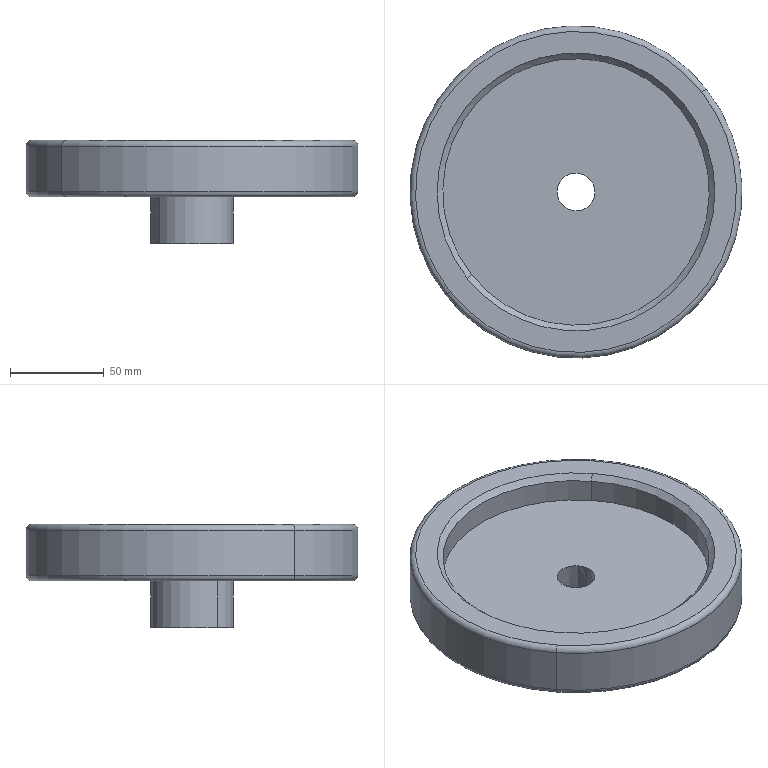Component | SolidWorks | 3-1 | 1 solid | 18 faces | box 177 x 177 x 55 mm | volume 506680 mm3 | cylinder 6 | cone 4 | torus 4 | plane 4 | commonest cylinder face diameters 177 x2 44 x2 142 x2
build123d program:
from build123d import *

# Parameters (mm, degrees)
CHAMFER1_SIZE = 3


with BuildPart() as part:
    # Sketch1 → Revolve1 (revolve)
    with BuildSketch(Plane(origin=(0, 0, 0), x_dir=(1, 0, 0), z_dir=(0, 1, 0))):
        with BuildLine():
            Line((0, 85.5), (0, 71))
            Line((0, 71), (15.508, 71))
            Line((15.508, 71), (15.508, 10.064))
            Line((15.508, 10.064), (55, 15))
            Line((55, 15), (55, 22))
            Line((55, 22), (30, 22))
            Line((30, 22), (30, 85.5))
            ThreePointArc((30, 85.5), (29.121, 87.621), (27, 88.5))
            Line((27, 88.5), (3, 88.5))
            ThreePointArc((3, 88.5), (0.8787, 87.621), (0, 85.5))
        make_face()
    revolve(axis=Axis((55, 0, 0), (-1, 0, 0)))

    # Chamfer1
    chamfer1_edges = [part.edges().sort_by_distance(p)[0] for p in [
        (0, 0, 71),
    ]]
    chamfer(chamfer1_edges, length=CHAMFER1_SIZE)


solid = part.part

# Placed as in the assembly
solid = solid.moved(Location((-135.043, 380.991, 857.751), (0, 90, 0)))
STEP:
#1=COLOUR_RGB('',0.7922,0.8196,0.9333);
#2=FILL_AREA_STYLE_COLOUR('',#1);
#3=FILL_AREA_STYLE('',(#2));
#4=SURFACE_STYLE_FILL_AREA(#3);
#5=SURFACE_SIDE_STYLE('',(#4));
#6=SURFACE_STYLE_USAGE(.BOTH.,#5);
#7=PRESENTATION_STYLE_ASSIGNMENT((#6));
#8=CARTESIAN_POINT('',(-7.51,13.267,33.652));
#9=VERTEX_POINT('',#8);
#10=CARTESIAN_POINT('',(-3.123,16.732,33.652));
#11=VERTEX_POINT('',#10);
#12=CARTESIAN_POINT('',(-5.317,15.,33.652));
#13=DIRECTION('',(0.,0.,1.));
#14=DIRECTION('',(-0.7848,-0.6197,0.));
#15=AXIS2_PLACEMENT_3D('',#12,#13,#14);
#16=CIRCLE('',#15,2.795);
#17=EDGE_CURVE('',#9,#11,#16,.T.);
#18=ORIENTED_EDGE('',*,*,#17,.F.);
#19=CARTESIAN_POINT('',(-7.603,13.194,33.77));
#20=VERTEX_POINT('',#19);
#21=CARTESIAN_POINT('',(-7.603,13.194,33.77));
#22=DIRECTION('',(-0.5549,-0.4382,0.7071));
#23=VECTOR('',#22,39.37);
#24=LINE('',#21,#23);
#25=EDGE_CURVE('',#9,#20,#24,.T.);
#26=ORIENTED_EDGE('',*,*,#25,.T.);
#27=CARTESIAN_POINT('',(-3.03,16.805,33.77));
#28=VERTEX_POINT('',#27);
#29=CARTESIAN_POINT('',(-5.317,15.,33.77));
#30=DIRECTION('',(-0.,-0.,-1.));
#31=DIRECTION('',(-0.7848,-0.6197,0.));
#32=AXIS2_PLACEMENT_3D('',#29,#30,#31);
#33=CIRCLE('',#32,2.913);
#34=EDGE_CURVE('',#28,#20,#33,.T.);
#35=ORIENTED_EDGE('',*,*,#34,.F.);
#36=CARTESIAN_POINT('',(-3.03,16.805,33.77));
#37=DIRECTION('',(0.5549,0.4382,0.7071));
#38=VECTOR('',#37,39.37);
#39=LINE('',#36,#38);
#40=EDGE_CURVE('',#11,#28,#39,.T.);
#41=ORIENTED_EDGE('',*,*,#40,.F.);
#42=EDGE_LOOP('',(#18,#26,#35,#41));
#43=FACE_OUTER_BOUND('',#42,.T.);
#44=CARTESIAN_POINT('',(-5.317,15.,33.77));
#45=DIRECTION('',(0.,0.,1.));
#46=DIRECTION('',(0.7848,0.6197,0.));
#47=AXIS2_PLACEMENT_3D('',#44,#45,#46);
#48=CONICAL_SURFACE('',#47,2.913,0.7854);
#49=ADVANCED_FACE('',(#43),#48,.F.);
#50=CARTESIAN_POINT('',(-8.051,12.84,33.652));
#51=VERTEX_POINT('',#50);
#52=CARTESIAN_POINT('',(-2.582,17.159,33.652));
#53=VERTEX_POINT('',#52);
#54=CARTESIAN_POINT('',(-5.317,15.,33.652));
#55=DIRECTION('',(-0.,-0.,-1.));
#56=DIRECTION('',(-0.7848,-0.6197,0.));
#57=AXIS2_PLACEMENT_3D('',#54,#55,#56);
#58=CIRCLE('',#57,3.484);
#59=EDGE_CURVE('',#51,#53,#58,.T.);
#60=ORIENTED_EDGE('',*,*,#59,.T.);
#61=CARTESIAN_POINT('',(-2.582,17.159,32.707));
#62=VERTEX_POINT('',#61);
#63=CARTESIAN_POINT('',(-2.582,17.159,31.604));
#64=DIRECTION('',(-0.,-0.,-1.));
#65=VECTOR('',#64,39.37);
#66=LINE('',#63,#65);
#67=EDGE_CURVE('',#53,#62,#66,.T.);
#68=ORIENTED_EDGE('',*,*,#67,.T.);
#69=CARTESIAN_POINT('',(-8.051,12.84,32.707));
#70=VERTEX_POINT('',#69);
#71=CARTESIAN_POINT('',(-5.317,15.,32.707));
#72=DIRECTION('',(-0.,-0.,-1.));
#73=DIRECTION('',(-0.7848,-0.6197,0.));
#74=AXIS2_PLACEMENT_3D('',#71,#72,#73);
#75=CIRCLE('',#74,3.484);
#76=EDGE_CURVE('',#70,#62,#75,.T.);
#77=ORIENTED_EDGE('',*,*,#76,.F.);
#78=CARTESIAN_POINT('',(-8.051,12.84,31.604));
#79=DIRECTION('',(-0.,-0.,-1.));
#80=VECTOR('',#79,39.37);
#81=LINE('',#78,#80);
#82=EDGE_CURVE('',#51,#70,#81,.T.);
#83=ORIENTED_EDGE('',*,*,#82,.F.);
#84=EDGE_LOOP('',(#60,#68,#77,#83));
#85=FACE_OUTER_BOUND('',#84,.T.);
#86=CARTESIAN_POINT('',(-5.317,15.,31.604));
#87=DIRECTION('',(-0.,-0.,-1.));
#88=DIRECTION('',(-0.7848,-0.6197,0.));
#89=AXIS2_PLACEMENT_3D('',#86,#87,#88);
#90=CYLINDRICAL_SURFACE('',#89,3.484);
#91=ADVANCED_FACE('',(#85),#90,.T.);
#92=ORIENTED_EDGE('',*,*,#76,.T.);
#93=CARTESIAN_POINT('',(-2.675,17.086,32.589));
#94=VERTEX_POINT('',#93);
#95=CARTESIAN_POINT('',(-2.675,17.086,32.707));
#96=DIRECTION('',(-0.6197,0.7848,-0.));
#97=DIRECTION('',(-0.7848,-0.6197,0.));
#98=AXIS2_PLACEMENT_3D('',#95,#96,#97);
#99=CIRCLE('',#98,0.1181);
#100=EDGE_CURVE('',#62,#94,#99,.T.);
#101=ORIENTED_EDGE('',*,*,#100,.T.);
#102=CARTESIAN_POINT('',(-7.958,12.914,32.589));
#103=VERTEX_POINT('',#102);
#104=CARTESIAN_POINT('',(-5.317,15.,32.589));
#105=DIRECTION('',(-0.,-0.,-1.));
#106=DIRECTION('',(-0.7848,-0.6197,0.));
#107=AXIS2_PLACEMENT_3D('',#104,#105,#106);
#108=CIRCLE('',#107,3.366);
#109=EDGE_CURVE('',#103,#94,#108,.T.);
#110=ORIENTED_EDGE('',*,*,#109,.F.);
#111=CARTESIAN_POINT('',(-7.958,12.914,32.707));
#112=DIRECTION('',(0.6197,-0.7848,0.));
#113=DIRECTION('',(0.7848,0.6197,0.));
#114=AXIS2_PLACEMENT_3D('',#111,#112,#113);
#115=CIRCLE('',#114,0.1181);
#116=EDGE_CURVE('',#70,#103,#115,.T.);
#117=ORIENTED_EDGE('',*,*,#116,.F.);
#118=EDGE_LOOP('',(#92,#101,#110,#117));
#119=FACE_OUTER_BOUND('',#118,.T.);
#120=CARTESIAN_POINT('',(-5.317,15.,32.707));
#121=DIRECTION('',(-0.,-0.,-1.));
#122=DIRECTION('',(-0.7848,-0.6197,0.));
#123=AXIS2_PLACEMENT_3D('',#120,#121,#122);
#124=TOROIDAL_SURFACE('',#123,3.366,0.1181);
#125=ADVANCED_FACE('',(#119),#124,.T.);
#126=CARTESIAN_POINT('',(-5.996,14.463,32.589));
#127=VERTEX_POINT('',#126);
#128=CARTESIAN_POINT('',(-4.637,15.536,32.589));
#129=VERTEX_POINT('',#128);
#130=CARTESIAN_POINT('',(-5.317,15.,32.589));
#131=DIRECTION('',(-0.,-0.,-1.));
#132=DIRECTION('',(-0.7848,-0.6197,0.));
#133=AXIS2_PLACEMENT_3D('',#130,#131,#132);
#134=CIRCLE('',#133,0.8661);
#135=EDGE_CURVE('',#127,#129,#134,.T.);
#136=ORIENTED_EDGE('',*,*,#135,.T.);
#137=CARTESIAN_POINT('',(-4.637,15.536,31.604));
#138=VERTEX_POINT('',#137);
#139=CARTESIAN_POINT('',(-4.637,15.536,31.604));
#140=DIRECTION('',(-0.,-0.,-1.));
#141=VECTOR('',#140,39.37);
#142=LINE('',#139,#141);
#143=EDGE_CURVE('',#129,#138,#142,.T.);
#144=ORIENTED_EDGE('',*,*,#143,.T.);
#145=CARTESIAN_POINT('',(-5.996,14.463,31.604));
#146=VERTEX_POINT('',#145);
#147=CARTESIAN_POINT('',(-5.317,15.,31.604));
#148=DIRECTION('',(-0.,-0.,-1.));
#149=DIRECTION('',(-0.7848,-0.6197,0.));
#150=AXIS2_PLACEMENT_3D('',#147,#148,#149);
#151=CIRCLE('',#150,0.8661);
#152=EDGE_CURVE('',#146,#138,#151,.T.);
#153=ORIENTED_EDGE('',*,*,#152,.F.);
#154=CARTESIAN_POINT('',(-5.996,14.463,31.604));
#155=DIRECTION('',(-0.,-0.,-1.));
#156=VECTOR('',#155,39.37);
#157=LINE('',#154,#156);
#158=EDGE_CURVE('',#127,#146,#157,.T.);
#159=ORIENTED_EDGE('',*,*,#158,.F.);
#160=EDGE_LOOP('',(#136,#144,#153,#159));
#161=FACE_OUTER_BOUND('',#160,.T.);
#162=CARTESIAN_POINT('',(-5.317,15.,31.604));
#163=DIRECTION('',(-0.,-0.,-1.));
#164=DIRECTION('',(-0.7848,-0.6197,0.));
#165=AXIS2_PLACEMENT_3D('',#162,#163,#164);
#166=CYLINDRICAL_SURFACE('',#165,0.8661);
#167=ADVANCED_FACE('',(#161),#166,.T.);
#168=CARTESIAN_POINT('',(-5.006,15.245,33.159));
#169=VERTEX_POINT('',#168);
#170=CARTESIAN_POINT('',(-5.628,14.754,33.159));
#171=VERTEX_POINT('',#170);
#172=CARTESIAN_POINT('',(-5.317,15.,33.159));
#173=DIRECTION('',(-0.,-0.,-1.));
#174=DIRECTION('',(-0.7848,-0.6197,0.));
#175=AXIS2_PLACEMENT_3D('',#172,#173,#174);
#176=CIRCLE('',#175,0.3962);
#177=EDGE_CURVE('',#169,#171,#176,.T.);
#178=ORIENTED_EDGE('',*,*,#177,.F.);
#179=CARTESIAN_POINT('',(-4.853,15.366,31.604));
#180=VERTEX_POINT('',#179);
#181=CARTESIAN_POINT('',(-4.853,15.366,31.604));
#182=DIRECTION('',(0.09734,0.07687,-0.9923));
#183=VECTOR('',#182,39.37);
#184=LINE('',#181,#183);
#185=EDGE_CURVE('',#169,#180,#184,.T.);
#186=ORIENTED_EDGE('',*,*,#185,.T.);
#187=CARTESIAN_POINT('',(-5.78,14.634,31.604));
#188=VERTEX_POINT('',#187);
#189=CARTESIAN_POINT('',(-5.317,15.,31.604));
#190=DIRECTION('',(-0.,-0.,-1.));
#191=DIRECTION('',(-0.7848,-0.6197,0.));
#192=AXIS2_PLACEMENT_3D('',#189,#190,#191);
#193=CIRCLE('',#192,0.5906);
#194=EDGE_CURVE('',#180,#188,#193,.T.);
#195=ORIENTED_EDGE('',*,*,#194,.T.);
#196=CARTESIAN_POINT('',(-5.78,14.634,31.604));
#197=DIRECTION('',(-0.09734,-0.07687,-0.9923));
#198=VECTOR('',#197,39.37);
#199=LINE('',#196,#198);
#200=EDGE_CURVE('',#171,#188,#199,.T.);
#201=ORIENTED_EDGE('',*,*,#200,.F.);
#202=EDGE_LOOP('',(#178,#186,#195,#201));
#203=FACE_OUTER_BOUND('',#202,.T.);
#204=CARTESIAN_POINT('',(-5.317,15.,31.604));
#205=DIRECTION('',(-0.,-0.,-1.));
#206=DIRECTION('',(-0.7848,-0.6197,0.));
#207=AXIS2_PLACEMENT_3D('',#204,#205,#206);
#208=CONICAL_SURFACE('',#207,0.5906,0.1244);
#209=ADVANCED_FACE('',(#203),#208,.F.);
#210=ORIENTED_EDGE('',*,*,#17,.T.);
#211=CARTESIAN_POINT('',(-3.123,16.732,33.159));
#212=VERTEX_POINT('',#211);
#213=CARTESIAN_POINT('',(-3.123,16.732,31.604));
#214=DIRECTION('',(-0.,-0.,-1.));
#215=VECTOR('',#214,39.37);
#216=LINE('',#213,#215);
#217=EDGE_CURVE('',#11,#212,#216,.T.);
#218=ORIENTED_EDGE('',*,*,#217,.T.);
#219=CARTESIAN_POINT('',(-7.51,13.267,33.159));
#220=VERTEX_POINT('',#219);
#221=CARTESIAN_POINT('',(-5.317,15.,33.159));
#222=DIRECTION('',(-0.,-0.,-1.));
#223=DIRECTION('',(-0.7848,-0.6197,0.));
#224=AXIS2_PLACEMENT_3D('',#221,#222,#223);
#225=CIRCLE('',#224,2.795);
#226=EDGE_CURVE('',#212,#220,#225,.T.);
#227=ORIENTED_EDGE('',*,*,#226,.T.);
#228=CARTESIAN_POINT('',(-7.51,13.267,31.604));
#229=DIRECTION('',(-0.,-0.,-1.));
#230=VECTOR('',#229,39.37);
#231=LINE('',#228,#230);
#232=EDGE_CURVE('',#9,#220,#231,.T.);
#233=ORIENTED_EDGE('',*,*,#232,.F.);
#234=EDGE_LOOP('',(#210,#218,#227,#233));
#235=FACE_OUTER_BOUND('',#234,.T.);
#236=CARTESIAN_POINT('',(-5.317,15.,31.604));
#237=DIRECTION('',(-0.,-0.,-1.));
#238=DIRECTION('',(-0.7848,-0.6197,0.));
#239=AXIS2_PLACEMENT_3D('',#236,#237,#238);
#240=CYLINDRICAL_SURFACE('',#239,2.795);
#241=ADVANCED_FACE('',(#235),#240,.F.);
#242=CARTESIAN_POINT('',(-7.958,12.914,33.77));
#243=VERTEX_POINT('',#242);
#244=CARTESIAN_POINT('',(-2.675,17.086,33.77));
#245=VERTEX_POINT('',#244);
#246=CARTESIAN_POINT('',(-5.317,15.,33.77));
#247=DIRECTION('',(-0.,-0.,-1.));
#248=DIRECTION('',(-0.7848,-0.6197,0.));
#249=AXIS2_PLACEMENT_3D('',#246,#247,#248);
#250=CIRCLE('',#249,3.366);
#251=EDGE_CURVE('',#243,#245,#250,.T.);
#252=ORIENTED_EDGE('',*,*,#251,.T.);
#253=CARTESIAN_POINT('',(-2.675,17.086,33.652));
#254=DIRECTION('',(-0.6197,0.7848,-0.));
#255=DIRECTION('',(-0.7848,-0.6197,0.));
#256=AXIS2_PLACEMENT_3D('',#253,#254,#255);
#257=CIRCLE('',#256,0.1181);
#258=EDGE_CURVE('',#245,#53,#257,.T.);
#259=ORIENTED_EDGE('',*,*,#258,.T.);
#260=ORIENTED_EDGE('',*,*,#59,.F.);
#261=CARTESIAN_POINT('',(-7.958,12.914,33.652));
#262=DIRECTION('',(0.6197,-0.7848,0.));
#263=DIRECTION('',(0.7848,0.6197,0.));
#264=AXIS2_PLACEMENT_3D('',#261,#262,#263);
#265=CIRCLE('',#264,0.1181);
#266=EDGE_CURVE('',#243,#51,#265,.T.);
#267=ORIENTED_EDGE('',*,*,#266,.F.);
#268=EDGE_LOOP('',(#252,#259,#260,#267));
#269=FACE_OUTER_BOUND('',#268,.T.);
#270=CARTESIAN_POINT('',(-5.317,15.,33.652));
#271=DIRECTION('',(-0.,-0.,-1.));
#272=DIRECTION('',(-0.7848,-0.6197,0.));
#273=AXIS2_PLACEMENT_3D('',#270,#271,#272);
#274=TOROIDAL_SURFACE('',#273,3.366,0.1181);
#275=ADVANCED_FACE('',(#269),#274,.T.);
#276=ORIENTED_EDGE('',*,*,#258,.F.);
#277=CARTESIAN_POINT('',(-5.317,15.,33.77));
#278=DIRECTION('',(-0.,-0.,-1.));
#279=DIRECTION('',(-0.7848,-0.6197,0.));
#280=AXIS2_PLACEMENT_3D('',#277,#278,#279);
#281=CIRCLE('',#280,3.366);
#282=EDGE_CURVE('',#245,#243,#281,.T.);
#283=ORIENTED_EDGE('',*,*,#282,.T.);
#284=ORIENTED_EDGE('',*,*,#266,.T.);
#285=CARTESIAN_POINT('',(-5.317,15.,33.652));
#286=DIRECTION('',(-0.,-0.,-1.));
#287=DIRECTION('',(-0.7848,-0.6197,0.));
#288=AXIS2_PLACEMENT_3D('',#285,#286,#287);
#289=CIRCLE('',#288,3.484);
#290=EDGE_CURVE('',#53,#51,#289,.T.);
#291=ORIENTED_EDGE('',*,*,#290,.F.);
#292=EDGE_LOOP('',(#276,#283,#284,#291));
#293=FACE_OUTER_BOUND('',#292,.T.);
#294=CARTESIAN_POINT('',(-5.317,15.,33.652));
#295=DIRECTION('',(-0.,-0.,-1.));
#296=DIRECTION('',(-0.7848,-0.6197,0.));
#297=AXIS2_PLACEMENT_3D('',#294,#295,#296);
#298=TOROIDAL_SURFACE('',#297,3.366,0.1181);
#299=ADVANCED_FACE('',(#293),#298,.T.);
#300=ORIENTED_EDGE('',*,*,#34,.T.);
#301=CARTESIAN_POINT('',(-5.317,15.,33.77));
#302=DIRECTION('',(-0.,-0.,-1.));
#303=DIRECTION('',(-0.7848,-0.6197,0.));
#304=AXIS2_PLACEMENT_3D('',#301,#302,#303);
#305=CIRCLE('',#304,2.913);
#306=EDGE_CURVE('',#20,#28,#305,.T.);
#307=ORIENTED_EDGE('',*,*,#306,.T.);
#308=EDGE_LOOP('',(#300,#307));
#309=FACE_BOUND('',#308,.T.);
#310=ORIENTED_EDGE('',*,*,#251,.F.);
#311=ORIENTED_EDGE('',*,*,#282,.F.);
#312=EDGE_LOOP('',(#310,#311));
#313=FACE_OUTER_BOUND('',#312,.T.);
#314=CARTESIAN_POINT('',(-5.317,15.,33.77));
#315=DIRECTION('',(-0.,-0.,-1.));
#316=DIRECTION('',(-0.7848,-0.6197,0.));
#317=AXIS2_PLACEMENT_3D('',#314,#315,#316);
#318=PLANE('',#317);
#319=ADVANCED_FACE('',(#309,#313),#318,.F.);
#320=ORIENTED_EDGE('',*,*,#217,.F.);
#321=CARTESIAN_POINT('',(-5.317,15.,33.652));
#322=DIRECTION('',(0.,0.,1.));
#323=DIRECTION('',(-0.7848,-0.6197,0.));
#324=AXIS2_PLACEMENT_3D('',#321,#322,#323);
#325=CIRCLE('',#324,2.795);
#326=EDGE_CURVE('',#11,#9,#325,.T.);
#327=ORIENTED_EDGE('',*,*,#326,.T.);
#328=ORIENTED_EDGE('',*,*,#232,.T.);
#329=CARTESIAN_POINT('',(-5.317,15.,33.159));
#330=DIRECTION('',(-0.,-0.,-1.));
#331=DIRECTION('',(-0.7848,-0.6197,0.));
#332=AXIS2_PLACEMENT_3D('',#329,#330,#331);
#333=CIRCLE('',#332,2.795);
#334=EDGE_CURVE('',#220,#212,#333,.T.);
#335=ORIENTED_EDGE('',*,*,#334,.T.);
#336=EDGE_LOOP('',(#320,#327,#328,#335));
#337=FACE_OUTER_BOUND('',#336,.T.);
#338=CARTESIAN_POINT('',(-5.317,15.,31.604));
#339=DIRECTION('',(-0.,-0.,-1.));
#340=DIRECTION('',(-0.7848,-0.6197,0.));
#341=AXIS2_PLACEMENT_3D('',#338,#339,#340);
#342=CYLINDRICAL_SURFACE('',#341,2.795);
#343=ADVANCED_FACE('',(#337),#342,.F.);
#344=CARTESIAN_POINT('',(-5.317,15.,33.159));
#345=DIRECTION('',(-0.,-0.,-1.));
#346=DIRECTION('',(-0.7848,-0.6197,0.));
#347=AXIS2_PLACEMENT_3D('',#344,#345,#346);
#348=CIRCLE('',#347,0.3962);
#349=EDGE_CURVE('',#171,#169,#348,.T.);
#350=ORIENTED_EDGE('',*,*,#349,.T.);
#351=ORIENTED_EDGE('',*,*,#177,.T.);
#352=EDGE_LOOP('',(#350,#351));
#353=FACE_BOUND('',#352,.T.);
#354=ORIENTED_EDGE('',*,*,#334,.F.);
#355=ORIENTED_EDGE('',*,*,#226,.F.);
#356=EDGE_LOOP('',(#354,#355));
#357=FACE_OUTER_BOUND('',#356,.T.);
#358=CARTESIAN_POINT('',(-5.317,15.,33.159));
#359=DIRECTION('',(0.,0.,1.));
#360=DIRECTION('',(0.7848,0.6197,-0.));
#361=AXIS2_PLACEMENT_3D('',#358,#359,#360);
#362=PLANE('',#361);
#363=ADVANCED_FACE('',(#353,#357),#362,.T.);
#364=ORIENTED_EDGE('',*,*,#185,.F.);
#365=ORIENTED_EDGE('',*,*,#349,.F.);
#366=ORIENTED_EDGE('',*,*,#200,.T.);
#367=CARTESIAN_POINT('',(-5.317,15.,31.604));
#368=DIRECTION('',(-0.,-0.,-1.));
#369=DIRECTION('',(-0.7848,-0.6197,0.));
#370=AXIS2_PLACEMENT_3D('',#367,#368,#369);
#371=CIRCLE('',#370,0.5906);
#372=EDGE_CURVE('',#188,#180,#371,.T.);
#373=ORIENTED_EDGE('',*,*,#372,.T.);
#374=EDGE_LOOP('',(#364,#365,#366,#373));
#375=FACE_OUTER_BOUND('',#374,.T.);
#376=CARTESIAN_POINT('',(-5.317,15.,31.604));
#377=DIRECTION('',(-0.,-0.,-1.));
#378=DIRECTION('',(-0.7848,-0.6197,0.));
#379=AXIS2_PLACEMENT_3D('',#376,#377,#378);
#380=CONICAL_SURFACE('',#379,0.5906,0.1244);
#381=ADVANCED_FACE('',(#375),#380,.F.);
#382=ORIENTED_EDGE('',*,*,#372,.F.);
#383=ORIENTED_EDGE('',*,*,#194,.F.);
#384=EDGE_LOOP('',(#382,#383));
#385=FACE_BOUND('',#384,.T.);
#386=ORIENTED_EDGE('',*,*,#152,.T.);
#387=CARTESIAN_POINT('',(-5.317,15.,31.604));
#388=DIRECTION('',(-0.,-0.,-1.));
#389=DIRECTION('',(-0.7848,-0.6197,0.));
#390=AXIS2_PLACEMENT_3D('',#387,#388,#389);
#391=CIRCLE('',#390,0.8661);
#392=EDGE_CURVE('',#138,#146,#391,.T.);
#393=ORIENTED_EDGE('',*,*,#392,.T.);
#394=EDGE_LOOP('',(#386,#393));
#395=FACE_OUTER_BOUND('',#394,.T.);
#396=CARTESIAN_POINT('',(-5.317,15.,31.604));
#397=DIRECTION('',(0.,0.,1.));
#398=DIRECTION('',(0.7848,0.6197,-0.));
#399=AXIS2_PLACEMENT_3D('',#396,#397,#398);
#400=PLANE('',#399);
#401=ADVANCED_FACE('',(#385,#395),#400,.F.);
#402=ORIENTED_EDGE('',*,*,#143,.F.);
#403=CARTESIAN_POINT('',(-5.317,15.,32.589));
#404=DIRECTION('',(-0.,-0.,-1.));
#405=DIRECTION('',(-0.7848,-0.6197,0.));
#406=AXIS2_PLACEMENT_3D('',#403,#404,#405);
#407=CIRCLE('',#406,0.8661);
#408=EDGE_CURVE('',#129,#127,#407,.T.);
#409=ORIENTED_EDGE('',*,*,#408,.T.);
#410=ORIENTED_EDGE('',*,*,#158,.T.);
#411=ORIENTED_EDGE('',*,*,#392,.F.);
#412=EDGE_LOOP('',(#402,#409,#410,#411));
#413=FACE_OUTER_BOUND('',#412,.T.);
#414=CARTESIAN_POINT('',(-5.317,15.,31.604));
#415=DIRECTION('',(-0.,-0.,-1.));
#416=DIRECTION('',(-0.7848,-0.6197,0.));
#417=AXIS2_PLACEMENT_3D('',#414,#415,#416);
#418=CYLINDRICAL_SURFACE('',#417,0.8661);
#419=ADVANCED_FACE('',(#413),#418,.T.);
#420=ORIENTED_EDGE('',*,*,#135,.F.);
#421=ORIENTED_EDGE('',*,*,#408,.F.);
#422=EDGE_LOOP('',(#420,#421));
#423=FACE_BOUND('',#422,.T.);
#424=ORIENTED_EDGE('',*,*,#109,.T.);
#425=CARTESIAN_POINT('',(-5.317,15.,32.589));
#426=DIRECTION('',(-0.,-0.,-1.));
#427=DIRECTION('',(-0.7848,-0.6197,0.));
#428=AXIS2_PLACEMENT_3D('',#425,#426,#427);
#429=CIRCLE('',#428,3.366);
#430=EDGE_CURVE('',#94,#103,#429,.T.);
#431=ORIENTED_EDGE('',*,*,#430,.T.);
#432=EDGE_LOOP('',(#424,#431));
#433=FACE_OUTER_BOUND('',#432,.T.);
#434=CARTESIAN_POINT('',(-5.317,15.,32.589));
#435=DIRECTION('',(0.,0.,1.));
#436=DIRECTION('',(0.7848,0.6197,-0.));
#437=AXIS2_PLACEMENT_3D('',#434,#435,#436);
#438=PLANE('',#437);
#439=ADVANCED_FACE('',(#423,#433),#438,.F.);
#440=ORIENTED_EDGE('',*,*,#100,.F.);
#441=CARTESIAN_POINT('',(-5.317,15.,32.707));
#442=DIRECTION('',(-0.,-0.,-1.));
#443=DIRECTION('',(-0.7848,-0.6197,0.));
#444=AXIS2_PLACEMENT_3D('',#441,#442,#443);
#445=CIRCLE('',#444,3.484);
#446=EDGE_CURVE('',#62,#70,#445,.T.);
#447=ORIENTED_EDGE('',*,*,#446,.T.);
#448=ORIENTED_EDGE('',*,*,#116,.T.);
#449=ORIENTED_EDGE('',*,*,#430,.F.);
#450=EDGE_LOOP('',(#440,#447,#448,#449));
#451=FACE_OUTER_BOUND('',#450,.T.);
#452=CARTESIAN_POINT('',(-5.317,15.,32.707));
#453=DIRECTION('',(-0.,-0.,-1.));
#454=DIRECTION('',(-0.7848,-0.6197,0.));
#455=AXIS2_PLACEMENT_3D('',#452,#453,#454);
#456=TOROIDAL_SURFACE('',#455,3.366,0.1181);
#457=ADVANCED_FACE('',(#451),#456,.T.);
#458=ORIENTED_EDGE('',*,*,#67,.F.);
#459=ORIENTED_EDGE('',*,*,#290,.T.);
#460=ORIENTED_EDGE('',*,*,#82,.T.);
#461=ORIENTED_EDGE('',*,*,#446,.F.);
#462=EDGE_LOOP('',(#458,#459,#460,#461));
#463=FACE_OUTER_BOUND('',#462,.T.);
#464=CARTESIAN_POINT('',(-5.317,15.,31.604));
#465=DIRECTION('',(-0.,-0.,-1.));
#466=DIRECTION('',(-0.7848,-0.6197,0.));
#467=AXIS2_PLACEMENT_3D('',#464,#465,#466);
#468=CYLINDRICAL_SURFACE('',#467,3.484);
#469=ADVANCED_FACE('',(#463),#468,.T.);
#470=ORIENTED_EDGE('',*,*,#25,.F.);
#471=ORIENTED_EDGE('',*,*,#326,.F.);
#472=ORIENTED_EDGE('',*,*,#40,.T.);
#473=ORIENTED_EDGE('',*,*,#306,.F.);
#474=EDGE_LOOP('',(#470,#471,#472,#473));
#475=FACE_OUTER_BOUND('',#474,.T.);
#476=CARTESIAN_POINT('',(-5.317,15.,33.77));
#477=DIRECTION('',(0.,0.,1.));
#478=DIRECTION('',(0.7848,0.6197,0.));
#479=AXIS2_PLACEMENT_3D('',#476,#477,#478);
#480=CONICAL_SURFACE('',#479,2.913,0.7854);
#481=ADVANCED_FACE('',(#475),#480,.F.);
#482=CLOSED_SHELL('',(#49,#91,#125,#167,#209,#241,#275,#299,#319,#343,#363,#381,#401,#419,#439,#457,#469,#481));
#483=MANIFOLD_SOLID_BREP('',#482);
#484=STYLED_ITEM('',(#7),#483);
#485=PRESENTATION_LAYER_ASSIGNMENT('','',(#484));
#486=(LENGTH_UNIT()NAMED_UNIT(*)SI_UNIT($,.METRE.));
#487=LENGTH_MEASURE_WITH_UNIT(LENGTH_MEASURE(0.0254),#486);
#488=DIMENSIONAL_EXPONENTS(1.,0.,0.,0.,0.,0.,0.);
#489=(CONVERSION_BASED_UNIT('',#487)LENGTH_UNIT()NAMED_UNIT(#488));
#490=UNCERTAINTY_MEASURE_WITH_UNIT(LENGTH_MEASURE(0.00001),#489,'','');
#491=(NAMED_UNIT(*)PLANE_ANGLE_UNIT()SI_UNIT($,.RADIAN.));
#492=(NAMED_UNIT(*)SI_UNIT($,.STERADIAN.)SOLID_ANGLE_UNIT());
#493=(GEOMETRIC_REPRESENTATION_CONTEXT(3)GLOBAL_UNCERTAINTY_ASSIGNED_CONTEXT((#490))GLOBAL_UNIT_ASSIGNED_CONTEXT((#489,#491,#492))REPRESENTATION_CONTEXT('',''));
#494=MECHANICAL_DESIGN_GEOMETRIC_PRESENTATION_REPRESENTATION('',(#484),#493);
#495=CARTESIAN_POINT('',(0.,0.,0.));
#496=DIRECTION('',(0.,0.,1.));
#497=DIRECTION('',(1.,0.,0.));
#498=AXIS2_PLACEMENT_3D('',#495,#496,#497);
#499=(LENGTH_UNIT()NAMED_UNIT(*)SI_UNIT($,.METRE.));
#500=LENGTH_MEASURE_WITH_UNIT(LENGTH_MEASURE(0.0254),#499);
#501=DIMENSIONAL_EXPONENTS(1.,0.,0.,0.,0.,0.,0.);
#502=(CONVERSION_BASED_UNIT('',#500)LENGTH_UNIT()NAMED_UNIT(#501));
#503=UNCERTAINTY_MEASURE_WITH_UNIT(LENGTH_MEASURE(0.00001),#502,'','');
#504=(NAMED_UNIT(*)PLANE_ANGLE_UNIT()SI_UNIT($,.RADIAN.));
#505=(NAMED_UNIT(*)SI_UNIT($,.STERADIAN.)SOLID_ANGLE_UNIT());
#506=(GEOMETRIC_REPRESENTATION_CONTEXT(3)GLOBAL_UNCERTAINTY_ASSIGNED_CONTEXT((#503))GLOBAL_UNIT_ASSIGNED_CONTEXT((#502,#504,#505))REPRESENTATION_CONTEXT('',''));
#507=ADVANCED_BREP_SHAPE_REPRESENTATION('',(#483,#498),#506);